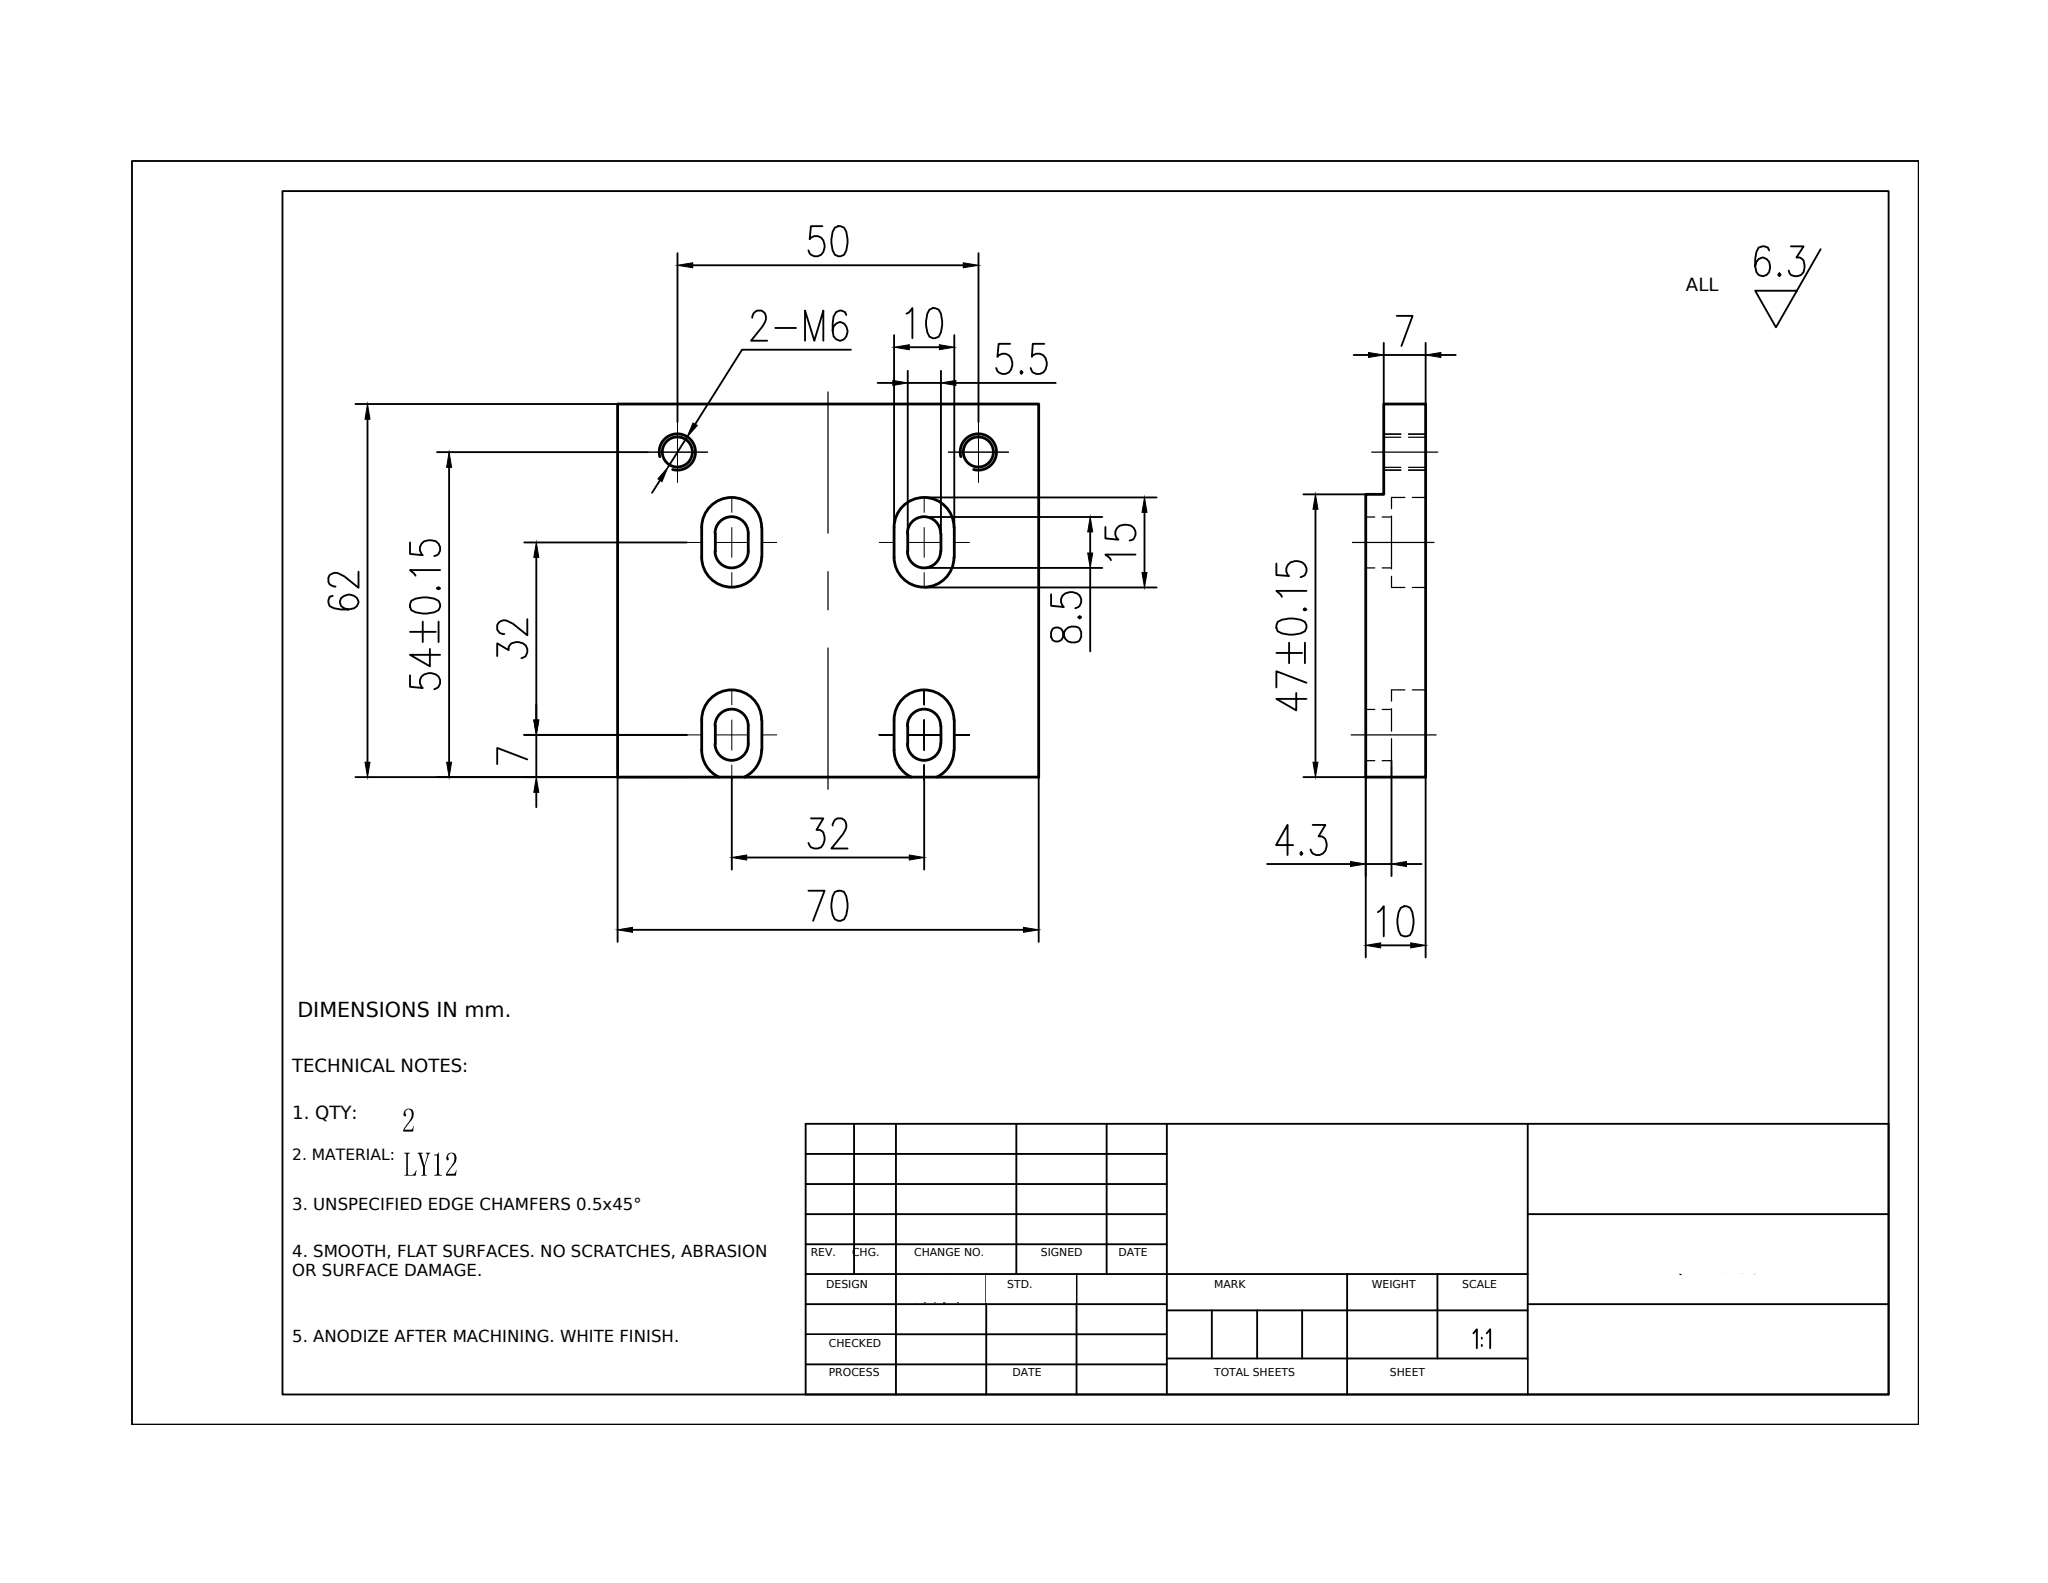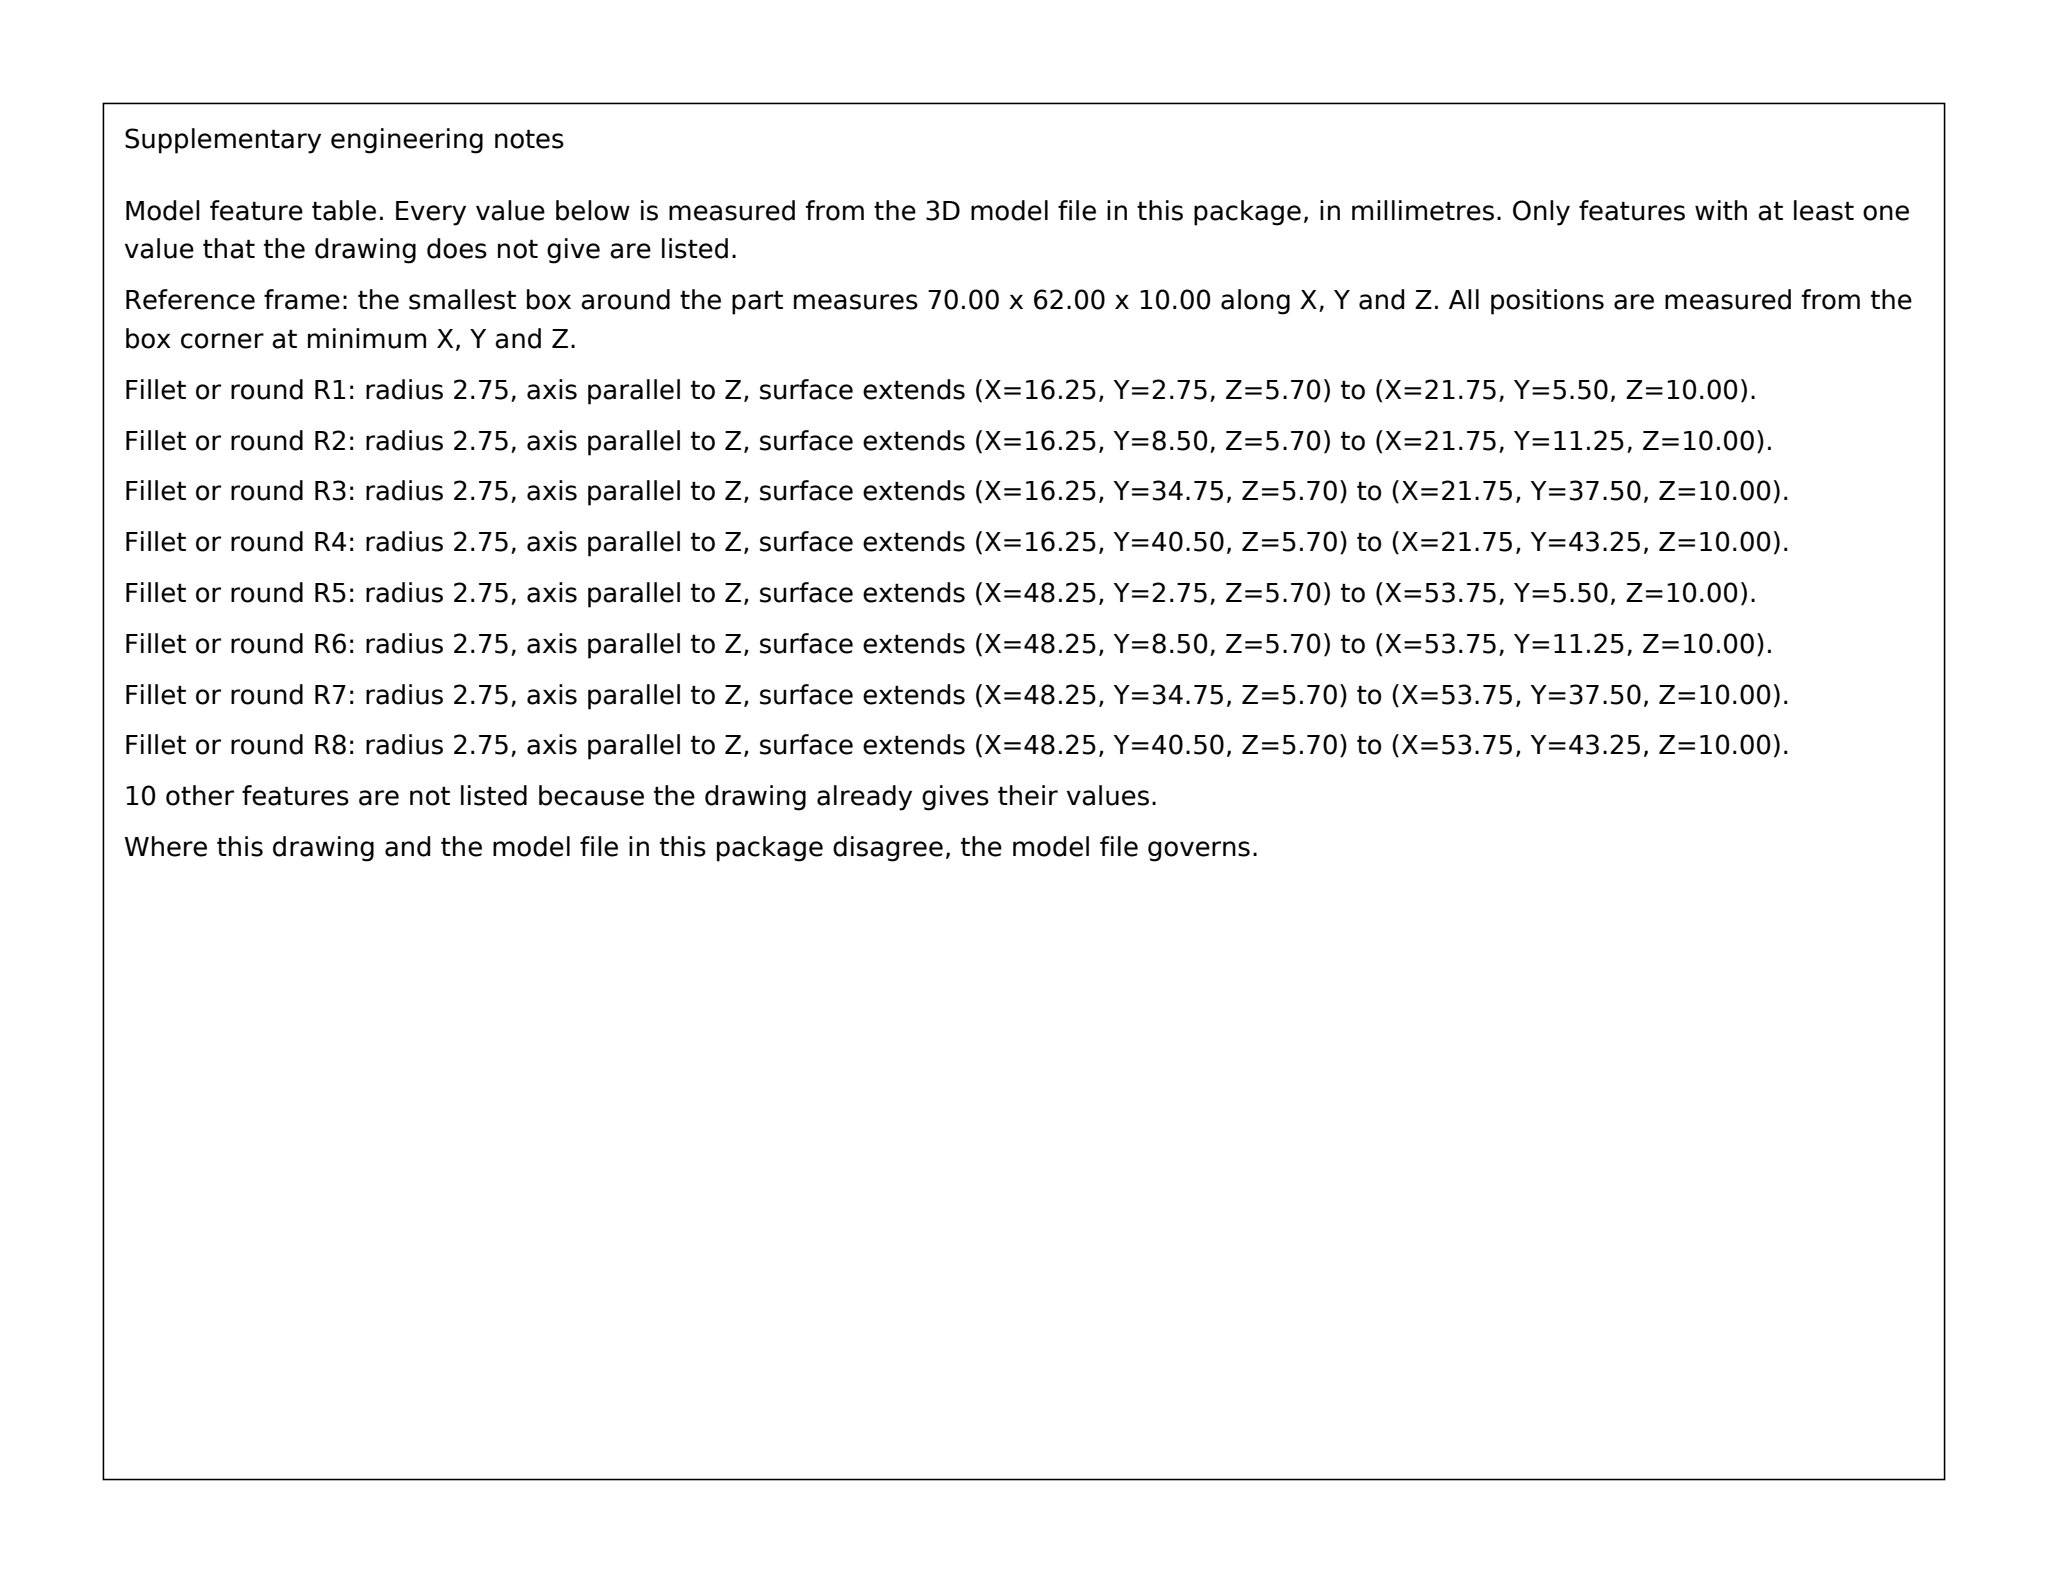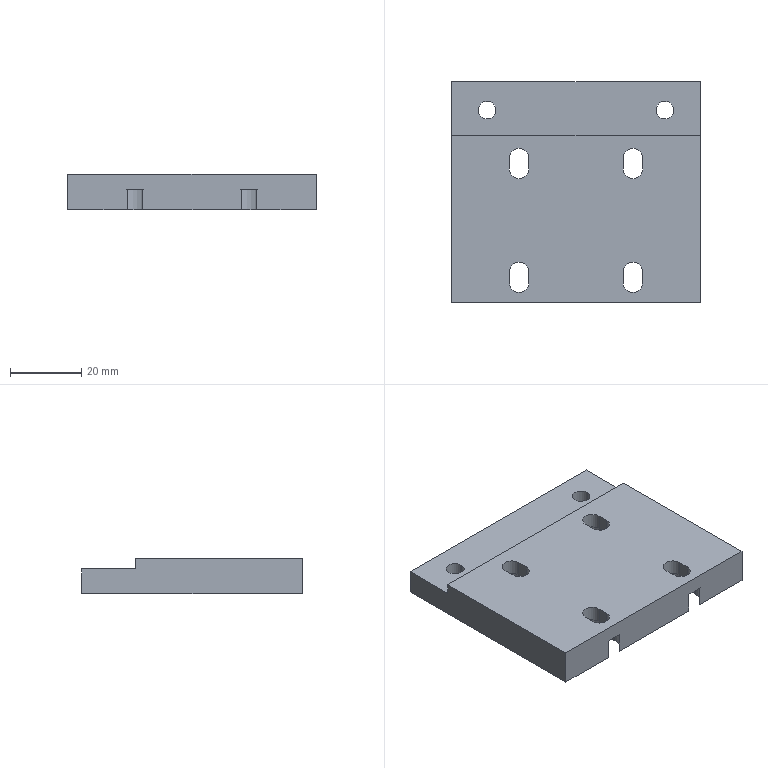Part | SolidWorks | mm | 1 solid | 50 faces | box 70 x 62 x 10 mm | volume 36369 mm3 | plane 28 | cylinder 22 | commonest cylinder face diameters 10 x10 5.5 x8 5 x4
build123d program:
from build123d import *

# Parameters (mm, degrees)
SKETCH1_W                                            = 70
SKETCH1_H                                            = 62
BOSS_EXTRUDE1_DEPTH                                  = 10
SKETCH2_W                                            = 70
SKETCH2_H                                            = 3
CUT_EXTRUDE1_DEPTH                                   = 15
HOLE_SIZE_ACCORDING_TO_THE_TYPE_OF_HEXAG_D           = 5.5
HOLE_SIZE_ACCORDING_TO_THE_TYPE_OF_HEXAG_CBORE_D     = 10
HOLE_SIZE_ACCORDING_TO_THE_TYPE_OF_HEXAG_CBORE_DEPTH = 5.7
M6_TAPPED_HOLE1_D                                    = 5
M6_TAPPED_HOLE1_DEPTH                                = 17
M6_TAPPED_HOLE1_TIP                                  = 1.502
CUT_EXTRUDE2_DEPTH                                   = 5.7
CUT_EXTRUDE3_DEPTH                                   = 48.101


with BuildPart() as part:
    # Sketch1 → Boss-Extrude1 (new body)
    with BuildSketch(Plane.XY):
        Rectangle(SKETCH1_W, SKETCH1_H)
    extrude(amount=BOSS_EXTRUDE1_DEPTH)

    # Sketch2 → Cut-Extrude1 (cut)
    with BuildSketch(Plane(origin=(0, 31, 0), x_dir=(1, 0, 0), z_dir=(0, 1, 0))):
        with Locations((0, -8.5)):
            Rectangle(SKETCH2_W, SKETCH2_H)
    extrude(amount=-CUT_EXTRUDE1_DEPTH, mode=Mode.SUBTRACT)

    # Hole Size according to the type of Hexag (through all)
    with Locations(Plane(origin=(-16, 8, 0), x_dir=(-1, 0, 0), z_dir=(0, 0, -1))):
        with Locations((0, 0), (-32, 0), (-32, -32), (0, -32)):
            CounterBoreHole(HOLE_SIZE_ACCORDING_TO_THE_TYPE_OF_HEXAG_D / 2, HOLE_SIZE_ACCORDING_TO_THE_TYPE_OF_HEXAG_CBORE_D / 2, HOLE_SIZE_ACCORDING_TO_THE_TYPE_OF_HEXAG_CBORE_DEPTH)

    # M6 Tapped Hole1
    with Locations(Plane(origin=(-25, 23, 7), x_dir=(1, 0, 0), z_dir=(0, 0, 1))):
        with Locations((0, 0), (50, 0)):
            Hole(M6_TAPPED_HOLE1_D / 2, depth=M6_TAPPED_HOLE1_DEPTH)
            with Locations((0, 0, -(M6_TAPPED_HOLE1_DEPTH + M6_TAPPED_HOLE1_TIP / 2))):  # 118° drill point
                Cone(0, M6_TAPPED_HOLE1_D / 2, M6_TAPPED_HOLE1_TIP, mode=Mode.SUBTRACT)

    # Sketch6 → Cut-Extrude2 (cut)
    with BuildSketch(Plane(origin=(0, 0, 0), x_dir=(-1, 0, 0), z_dir=(0, 0, -1))):
        with BuildLine():
            Line((-21, 5.5), (-21, 10.5))
            ThreePointArc((-21, 10.5), (-16, 15.5), (-11, 10.5))
            Line((-11, 10.5), (-11, 5.5))
            ThreePointArc((-11, 5.5), (-16, 0.5), (-21, 5.5))
        make_face()
        with BuildLine():
            Line((-11, -21.5), (-11, -26.5))
            ThreePointArc((-11, -26.5), (-16, -31.5), (-21, -26.5))
            Line((-21, -26.5), (-21, -21.5))
            ThreePointArc((-21, -21.5), (-16, -16.5), (-11, -21.5))
        make_face()
        with BuildLine():
            Line((11, -21.5), (11, -26.5))
            ThreePointArc((11, -26.5), (16, -31.5), (21, -26.5))
            Line((21, -26.5), (21, -21.5))
            ThreePointArc((21, -21.5), (16, -16.5), (11, -21.5))
        make_face()
        with BuildLine():
            Line((21, 5.5), (21, 10.5))
            ThreePointArc((21, 10.5), (16, 15.5), (11, 10.5))
            Line((11, 10.5), (11, 5.5))
            ThreePointArc((11, 5.5), (16, 0.5), (21, 5.5))
        make_face()
    extrude(amount=-CUT_EXTRUDE2_DEPTH, mode=Mode.SUBTRACT)

    # Sketch7 → Cut-Extrude3 (cut, through all)
    with BuildSketch(Plane(origin=(0, 0, 5.7), x_dir=(-1, 0, 0), z_dir=(0, 0, -1))):
        with BuildLine():
            Line((-13.25, 9.5), (-13.25, 6.5))
            ThreePointArc((-13.25, 6.5), (-16, 3.75), (-18.75, 6.5))
            Line((-18.75, 6.5), (-18.75, 9.5))
            ThreePointArc((-18.75, 9.5), (-16, 12.25), (-13.25, 9.5))
        make_face()
        with BuildLine():
            Line((-13.25, -25.5), (-13.25, -22.5))
            ThreePointArc((-13.25, -22.5), (-16, -19.75), (-18.75, -22.5))
            Line((-18.75, -22.5), (-18.75, -25.5))
            ThreePointArc((-18.75, -25.5), (-16, -28.25), (-13.25, -25.5))
        make_face()
        with BuildLine():
            Line((13.25, -25.5), (13.25, -22.5))
            ThreePointArc((13.25, -22.5), (16, -19.75), (18.75, -22.5))
            Line((18.75, -22.5), (18.75, -25.5))
            ThreePointArc((18.75, -25.5), (16, -28.25), (13.25, -25.5))
        make_face()
        with BuildLine():
            Line((13.25, 9.5), (13.25, 6.5))
            ThreePointArc((13.25, 6.5), (16, 3.75), (18.75, 6.5))
            Line((18.75, 6.5), (18.75, 9.5))
            ThreePointArc((18.75, 9.5), (16, 12.25), (13.25, 9.5))
        make_face()
    extrude(amount=-CUT_EXTRUDE3_DEPTH, mode=Mode.SUBTRACT)


solid = part.part